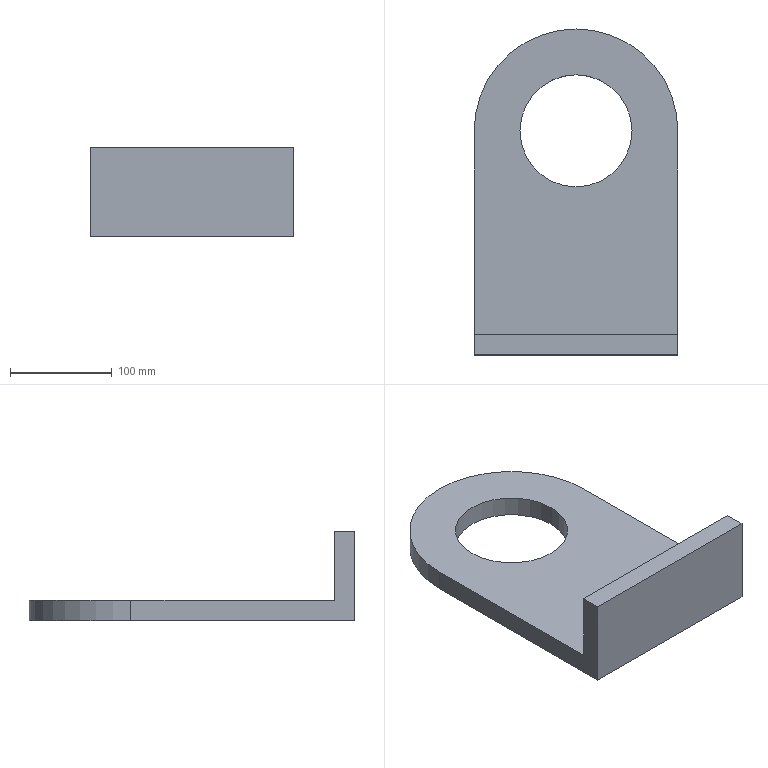Component | SolidWorks | MotorMount-1 | 1 solid | 10 faces | box 200 x 320 x 88 mm | volume 1276093 mm3 | plane 7 | cylinder 3 | commonest cylinder face diameters 110 x2 200 x1 | material 45
build123d program:
from build123d import *

# Parameters (mm, degrees)
SKETCH1_R           = 55
BOSS_EXTRUDE1_DEPTH = 20
SKETCH2_W           = 200
SKETCH2_H           = 88
BOSS_EXTRUDE2_DEPTH = 20


with BuildPart() as part:
    # Sketch1 → Boss-Extrude1 (new body)
    with BuildSketch(Plane.XY):
        with BuildLine():
            Line((-100, 0), (-100, -200))
            Line((-100, -200), (100, -200))
            Line((100, -200), (100, 0))
            ThreePointArc((100, 0), (0, 100), (-100, 0))
        make_face()
        Circle(SKETCH1_R, mode=Mode.SUBTRACT)
    extrude(amount=BOSS_EXTRUDE1_DEPTH)

    # Sketch2 → Boss-Extrude2 (add)
    with BuildSketch(Plane.XZ.offset(200)):
        with Locations((0, 44)):
            Rectangle(SKETCH2_W, SKETCH2_H)
    extrude(amount=BOSS_EXTRUDE2_DEPTH)


solid = part.part

# Placed as in the assembly
solid = solid.moved(Location((110.202, 126.699, 514.267), (0, 0, 0)))
STEP:
#1=COLOUR_RGB('',0.7922,0.8196,0.9333);
#2=FILL_AREA_STYLE_COLOUR('',#1);
#3=FILL_AREA_STYLE('',(#2));
#4=SURFACE_STYLE_FILL_AREA(#3);
#5=SURFACE_SIDE_STYLE('',(#4));
#6=SURFACE_STYLE_USAGE(.BOTH.,#5);
#7=PRESENTATION_STYLE_ASSIGNMENT((#6));
#8=CARTESIAN_POINT('',(2.173,4.988,21.034));
#9=VERTEX_POINT('',#8);
#10=CARTESIAN_POINT('',(6.504,4.988,21.034));
#11=VERTEX_POINT('',#10);
#12=CARTESIAN_POINT('',(4.339,4.988,21.034));
#13=DIRECTION('',(0.,0.,1.));
#14=DIRECTION('',(1.,0.,0.));
#15=AXIS2_PLACEMENT_3D('',#12,#13,#14);
#16=CIRCLE('',#15,2.165);
#17=EDGE_CURVE('',#9,#11,#16,.T.);
#18=ORIENTED_EDGE('',*,*,#17,.T.);
#19=CARTESIAN_POINT('',(6.504,4.988,20.247));
#20=VERTEX_POINT('',#19);
#21=CARTESIAN_POINT('',(6.504,4.988,21.034));
#22=DIRECTION('',(0.,0.,-1.));
#23=VECTOR('',#22,39.37);
#24=LINE('',#21,#23);
#25=EDGE_CURVE('',#11,#20,#24,.T.);
#26=ORIENTED_EDGE('',*,*,#25,.T.);
#27=CARTESIAN_POINT('',(2.173,4.988,20.247));
#28=VERTEX_POINT('',#27);
#29=CARTESIAN_POINT('',(4.339,4.988,20.247));
#30=DIRECTION('',(0.,0.,1.));
#31=DIRECTION('',(1.,0.,0.));
#32=AXIS2_PLACEMENT_3D('',#29,#30,#31);
#33=CIRCLE('',#32,2.165);
#34=EDGE_CURVE('',#28,#20,#33,.T.);
#35=ORIENTED_EDGE('',*,*,#34,.F.);
#36=CARTESIAN_POINT('',(2.173,4.988,21.034));
#37=DIRECTION('',(0.,0.,-1.));
#38=VECTOR('',#37,39.37);
#39=LINE('',#36,#38);
#40=EDGE_CURVE('',#9,#28,#39,.T.);
#41=ORIENTED_EDGE('',*,*,#40,.F.);
#42=EDGE_LOOP('',(#18,#26,#35,#41));
#43=FACE_OUTER_BOUND('',#42,.T.);
#44=CARTESIAN_POINT('',(4.339,4.988,21.034));
#45=DIRECTION('',(0.,0.,-1.));
#46=DIRECTION('',(-1.,0.,0.));
#47=AXIS2_PLACEMENT_3D('',#44,#45,#46);
#48=CYLINDRICAL_SURFACE('',#47,2.165);
#49=ADVANCED_FACE('',(#43),#48,.F.);
#50=CARTESIAN_POINT('',(8.276,4.988,21.034));
#51=VERTEX_POINT('',#50);
#52=CARTESIAN_POINT('',(0.4017,4.988,21.034));
#53=VERTEX_POINT('',#52);
#54=CARTESIAN_POINT('',(4.339,4.988,21.034));
#55=DIRECTION('',(0.,0.,1.));
#56=DIRECTION('',(1.,0.,0.));
#57=AXIS2_PLACEMENT_3D('',#54,#55,#56);
#58=CIRCLE('',#57,3.937);
#59=EDGE_CURVE('',#51,#53,#58,.T.);
#60=ORIENTED_EDGE('',*,*,#59,.T.);
#61=CARTESIAN_POINT('',(0.4017,-2.886,21.034));
#62=VERTEX_POINT('',#61);
#63=CARTESIAN_POINT('',(0.4017,4.988,21.034));
#64=DIRECTION('',(0.,-1.,0.));
#65=VECTOR('',#64,39.37);
#66=LINE('',#63,#65);
#67=EDGE_CURVE('',#53,#62,#66,.T.);
#68=ORIENTED_EDGE('',*,*,#67,.T.);
#69=CARTESIAN_POINT('',(8.276,-2.886,21.034));
#70=VERTEX_POINT('',#69);
#71=CARTESIAN_POINT('',(0.4017,-2.886,21.034));
#72=DIRECTION('',(1.,0.,0.));
#73=VECTOR('',#72,39.37);
#74=LINE('',#71,#73);
#75=EDGE_CURVE('',#62,#70,#74,.T.);
#76=ORIENTED_EDGE('',*,*,#75,.T.);
#77=CARTESIAN_POINT('',(8.276,-2.886,21.034));
#78=DIRECTION('',(0.,1.,0.));
#79=VECTOR('',#78,39.37);
#80=LINE('',#77,#79);
#81=EDGE_CURVE('',#70,#51,#80,.T.);
#82=ORIENTED_EDGE('',*,*,#81,.T.);
#83=EDGE_LOOP('',(#60,#68,#76,#82));
#84=FACE_OUTER_BOUND('',#83,.T.);
#85=ORIENTED_EDGE('',*,*,#17,.F.);
#86=CARTESIAN_POINT('',(4.339,4.988,21.034));
#87=DIRECTION('',(0.,0.,1.));
#88=DIRECTION('',(1.,0.,0.));
#89=AXIS2_PLACEMENT_3D('',#86,#87,#88);
#90=CIRCLE('',#89,2.165);
#91=EDGE_CURVE('',#11,#9,#90,.T.);
#92=ORIENTED_EDGE('',*,*,#91,.F.);
#93=EDGE_LOOP('',(#85,#92));
#94=FACE_BOUND('',#93,.T.);
#95=CARTESIAN_POINT('',(4.339,4.988,21.034));
#96=DIRECTION('',(0.,0.,1.));
#97=DIRECTION('',(1.,0.,0.));
#98=AXIS2_PLACEMENT_3D('',#95,#96,#97);
#99=PLANE('',#98);
#100=ADVANCED_FACE('',(#84,#94),#99,.T.);
#101=CARTESIAN_POINT('',(8.276,4.988,20.247));
#102=VERTEX_POINT('',#101);
#103=CARTESIAN_POINT('',(0.4017,4.988,20.247));
#104=VERTEX_POINT('',#103);
#105=CARTESIAN_POINT('',(4.339,4.988,20.247));
#106=DIRECTION('',(0.,0.,1.));
#107=DIRECTION('',(1.,0.,0.));
#108=AXIS2_PLACEMENT_3D('',#105,#106,#107);
#109=CIRCLE('',#108,3.937);
#110=EDGE_CURVE('',#102,#104,#109,.T.);
#111=ORIENTED_EDGE('',*,*,#110,.F.);
#112=CARTESIAN_POINT('',(8.276,-3.673,20.247));
#113=VERTEX_POINT('',#112);
#114=CARTESIAN_POINT('',(8.276,-2.886,20.247));
#115=DIRECTION('',(0.,1.,0.));
#116=VECTOR('',#115,39.37);
#117=LINE('',#114,#116);
#118=EDGE_CURVE('',#113,#102,#117,.T.);
#119=ORIENTED_EDGE('',*,*,#118,.F.);
#120=CARTESIAN_POINT('',(0.4017,-3.673,20.247));
#121=VERTEX_POINT('',#120);
#122=CARTESIAN_POINT('',(0.4017,-3.673,20.247));
#123=DIRECTION('',(1.,0.,0.));
#124=VECTOR('',#123,39.37);
#125=LINE('',#122,#124);
#126=EDGE_CURVE('',#121,#113,#125,.T.);
#127=ORIENTED_EDGE('',*,*,#126,.F.);
#128=CARTESIAN_POINT('',(0.4017,4.988,20.247));
#129=DIRECTION('',(0.,-1.,0.));
#130=VECTOR('',#129,39.37);
#131=LINE('',#128,#130);
#132=EDGE_CURVE('',#104,#121,#131,.T.);
#133=ORIENTED_EDGE('',*,*,#132,.F.);
#134=EDGE_LOOP('',(#111,#119,#127,#133));
#135=FACE_OUTER_BOUND('',#134,.T.);
#136=ORIENTED_EDGE('',*,*,#34,.T.);
#137=CARTESIAN_POINT('',(4.339,4.988,20.247));
#138=DIRECTION('',(0.,0.,1.));
#139=DIRECTION('',(1.,0.,0.));
#140=AXIS2_PLACEMENT_3D('',#137,#138,#139);
#141=CIRCLE('',#140,2.165);
#142=EDGE_CURVE('',#20,#28,#141,.T.);
#143=ORIENTED_EDGE('',*,*,#142,.T.);
#144=EDGE_LOOP('',(#136,#143));
#145=FACE_BOUND('',#144,.T.);
#146=CARTESIAN_POINT('',(4.339,4.988,20.247));
#147=DIRECTION('',(0.,0.,1.));
#148=DIRECTION('',(1.,0.,0.));
#149=AXIS2_PLACEMENT_3D('',#146,#147,#148);
#150=PLANE('',#149);
#151=ADVANCED_FACE('',(#135,#145),#150,.F.);
#152=ORIENTED_EDGE('',*,*,#110,.T.);
#153=CARTESIAN_POINT('',(0.4017,4.988,21.034));
#154=DIRECTION('',(0.,0.,-1.));
#155=VECTOR('',#154,39.37);
#156=LINE('',#153,#155);
#157=EDGE_CURVE('',#53,#104,#156,.T.);
#158=ORIENTED_EDGE('',*,*,#157,.F.);
#159=ORIENTED_EDGE('',*,*,#59,.F.);
#160=CARTESIAN_POINT('',(8.276,4.988,21.034));
#161=DIRECTION('',(0.,0.,-1.));
#162=VECTOR('',#161,39.37);
#163=LINE('',#160,#162);
#164=EDGE_CURVE('',#51,#102,#163,.T.);
#165=ORIENTED_EDGE('',*,*,#164,.T.);
#166=EDGE_LOOP('',(#152,#158,#159,#165));
#167=FACE_OUTER_BOUND('',#166,.T.);
#168=CARTESIAN_POINT('',(4.339,4.988,21.034));
#169=DIRECTION('',(0.,0.,-1.));
#170=DIRECTION('',(-1.,0.,0.));
#171=AXIS2_PLACEMENT_3D('',#168,#169,#170);
#172=CYLINDRICAL_SURFACE('',#171,3.937);
#173=ADVANCED_FACE('',(#167),#172,.T.);
#174=ORIENTED_EDGE('',*,*,#132,.T.);
#175=CARTESIAN_POINT('',(0.4017,-3.673,23.711));
#176=VERTEX_POINT('',#175);
#177=CARTESIAN_POINT('',(0.4017,-3.673,20.247));
#178=DIRECTION('',(0.,0.,-1.));
#179=VECTOR('',#178,39.37);
#180=LINE('',#177,#179);
#181=EDGE_CURVE('',#176,#121,#180,.T.);
#182=ORIENTED_EDGE('',*,*,#181,.F.);
#183=CARTESIAN_POINT('',(0.4017,-2.886,23.711));
#184=VERTEX_POINT('',#183);
#185=CARTESIAN_POINT('',(0.4017,-3.673,23.711));
#186=DIRECTION('',(0.,1.,0.));
#187=VECTOR('',#186,39.37);
#188=LINE('',#185,#187);
#189=EDGE_CURVE('',#176,#184,#188,.T.);
#190=ORIENTED_EDGE('',*,*,#189,.T.);
#191=CARTESIAN_POINT('',(0.4017,-2.886,20.247));
#192=DIRECTION('',(0.,0.,-1.));
#193=VECTOR('',#192,39.37);
#194=LINE('',#191,#193);
#195=EDGE_CURVE('',#184,#62,#194,.T.);
#196=ORIENTED_EDGE('',*,*,#195,.T.);
#197=ORIENTED_EDGE('',*,*,#67,.F.);
#198=ORIENTED_EDGE('',*,*,#157,.T.);
#199=EDGE_LOOP('',(#174,#182,#190,#196,#197,#198));
#200=FACE_OUTER_BOUND('',#199,.T.);
#201=CARTESIAN_POINT('',(0.4017,4.988,21.034));
#202=DIRECTION('',(1.,0.,0.));
#203=DIRECTION('',(-0.,1.,0.));
#204=AXIS2_PLACEMENT_3D('',#201,#202,#203);
#205=PLANE('',#204);
#206=ADVANCED_FACE('',(#200),#205,.F.);
#207=ORIENTED_EDGE('',*,*,#118,.T.);
#208=ORIENTED_EDGE('',*,*,#164,.F.);
#209=ORIENTED_EDGE('',*,*,#81,.F.);
#210=CARTESIAN_POINT('',(8.276,-2.886,23.711));
#211=VERTEX_POINT('',#210);
#212=CARTESIAN_POINT('',(8.276,-2.886,20.247));
#213=DIRECTION('',(0.,0.,1.));
#214=VECTOR('',#213,39.37);
#215=LINE('',#212,#214);
#216=EDGE_CURVE('',#70,#211,#215,.T.);
#217=ORIENTED_EDGE('',*,*,#216,.T.);
#218=CARTESIAN_POINT('',(8.276,-3.673,23.711));
#219=VERTEX_POINT('',#218);
#220=CARTESIAN_POINT('',(8.276,-3.673,23.711));
#221=DIRECTION('',(0.,1.,0.));
#222=VECTOR('',#221,39.37);
#223=LINE('',#220,#222);
#224=EDGE_CURVE('',#219,#211,#223,.T.);
#225=ORIENTED_EDGE('',*,*,#224,.F.);
#226=CARTESIAN_POINT('',(8.276,-3.673,20.247));
#227=DIRECTION('',(0.,0.,1.));
#228=VECTOR('',#227,39.37);
#229=LINE('',#226,#228);
#230=EDGE_CURVE('',#113,#219,#229,.T.);
#231=ORIENTED_EDGE('',*,*,#230,.F.);
#232=EDGE_LOOP('',(#207,#208,#209,#217,#225,#231));
#233=FACE_OUTER_BOUND('',#232,.T.);
#234=CARTESIAN_POINT('',(8.276,-2.886,21.034));
#235=DIRECTION('',(-1.,0.,0.));
#236=DIRECTION('',(-0.,-1.,0.));
#237=AXIS2_PLACEMENT_3D('',#234,#235,#236);
#238=PLANE('',#237);
#239=ADVANCED_FACE('',(#233),#238,.F.);
#240=ORIENTED_EDGE('',*,*,#25,.F.);
#241=ORIENTED_EDGE('',*,*,#91,.T.);
#242=ORIENTED_EDGE('',*,*,#40,.T.);
#243=ORIENTED_EDGE('',*,*,#142,.F.);
#244=EDGE_LOOP('',(#240,#241,#242,#243));
#245=FACE_OUTER_BOUND('',#244,.T.);
#246=CARTESIAN_POINT('',(4.339,4.988,21.034));
#247=DIRECTION('',(0.,0.,-1.));
#248=DIRECTION('',(-1.,0.,0.));
#249=AXIS2_PLACEMENT_3D('',#246,#247,#248);
#250=CYLINDRICAL_SURFACE('',#249,2.165);
#251=ADVANCED_FACE('',(#245),#250,.F.);
#252=ORIENTED_EDGE('',*,*,#75,.F.);
#253=ORIENTED_EDGE('',*,*,#195,.F.);
#254=CARTESIAN_POINT('',(0.4017,-2.886,23.711));
#255=DIRECTION('',(-1.,0.,0.));
#256=VECTOR('',#255,39.37);
#257=LINE('',#254,#256);
#258=EDGE_CURVE('',#211,#184,#257,.T.);
#259=ORIENTED_EDGE('',*,*,#258,.F.);
#260=ORIENTED_EDGE('',*,*,#216,.F.);
#261=EDGE_LOOP('',(#252,#253,#259,#260));
#262=FACE_OUTER_BOUND('',#261,.T.);
#263=CARTESIAN_POINT('',(4.339,-2.886,20.247));
#264=DIRECTION('',(0.,1.,0.));
#265=DIRECTION('',(0.,0.,1.));
#266=AXIS2_PLACEMENT_3D('',#263,#264,#265);
#267=PLANE('',#266);
#268=ADVANCED_FACE('',(#262),#267,.T.);
#269=ORIENTED_EDGE('',*,*,#258,.T.);
#270=ORIENTED_EDGE('',*,*,#189,.F.);
#271=CARTESIAN_POINT('',(0.4017,-3.673,23.711));
#272=DIRECTION('',(-1.,0.,0.));
#273=VECTOR('',#272,39.37);
#274=LINE('',#271,#273);
#275=EDGE_CURVE('',#219,#176,#274,.T.);
#276=ORIENTED_EDGE('',*,*,#275,.F.);
#277=ORIENTED_EDGE('',*,*,#224,.T.);
#278=EDGE_LOOP('',(#269,#270,#276,#277));
#279=FACE_OUTER_BOUND('',#278,.T.);
#280=CARTESIAN_POINT('',(0.4017,-3.673,23.711));
#281=DIRECTION('',(0.,0.,-1.));
#282=DIRECTION('',(-1.,0.,0.));
#283=AXIS2_PLACEMENT_3D('',#280,#281,#282);
#284=PLANE('',#283);
#285=ADVANCED_FACE('',(#279),#284,.F.);
#286=ORIENTED_EDGE('',*,*,#181,.T.);
#287=ORIENTED_EDGE('',*,*,#126,.T.);
#288=ORIENTED_EDGE('',*,*,#230,.T.);
#289=ORIENTED_EDGE('',*,*,#275,.T.);
#290=EDGE_LOOP('',(#286,#287,#288,#289));
#291=FACE_OUTER_BOUND('',#290,.T.);
#292=CARTESIAN_POINT('',(4.339,-3.673,20.247));
#293=DIRECTION('',(0.,1.,0.));
#294=DIRECTION('',(0.,0.,1.));
#295=AXIS2_PLACEMENT_3D('',#292,#293,#294);
#296=PLANE('',#295);
#297=ADVANCED_FACE('',(#291),#296,.F.);
#298=CLOSED_SHELL('',(#49,#100,#151,#173,#206,#239,#251,#268,#285,#297));
#299=MANIFOLD_SOLID_BREP('',#298);
#300=STYLED_ITEM('',(#7),#299);
#301=(LENGTH_UNIT()NAMED_UNIT(*)SI_UNIT($,.METRE.));
#302=LENGTH_MEASURE_WITH_UNIT(LENGTH_MEASURE(0.0254),#301);
#303=DIMENSIONAL_EXPONENTS(1.,0.,0.,0.,0.,0.,0.);
#304=(CONVERSION_BASED_UNIT('',#302)LENGTH_UNIT()NAMED_UNIT(#303));
#305=UNCERTAINTY_MEASURE_WITH_UNIT(LENGTH_MEASURE(0.00001),#304,'','');
#306=(NAMED_UNIT(*)PLANE_ANGLE_UNIT()SI_UNIT($,.RADIAN.));
#307=(NAMED_UNIT(*)SI_UNIT($,.STERADIAN.)SOLID_ANGLE_UNIT());
#308=(GEOMETRIC_REPRESENTATION_CONTEXT(3)GLOBAL_UNCERTAINTY_ASSIGNED_CONTEXT((#305))GLOBAL_UNIT_ASSIGNED_CONTEXT((#304,#306,#307))REPRESENTATION_CONTEXT('',''));
#309=MECHANICAL_DESIGN_GEOMETRIC_PRESENTATION_REPRESENTATION('',(#300),#308);
#310=PRESENTATION_LAYER_ASSIGNMENT('','',(#300));
#311=CARTESIAN_POINT('',(0.,0.,0.));
#312=DIRECTION('',(0.,0.,1.));
#313=DIRECTION('',(1.,0.,0.));
#314=AXIS2_PLACEMENT_3D('',#311,#312,#313);
#315=(LENGTH_UNIT()NAMED_UNIT(*)SI_UNIT($,.METRE.));
#316=LENGTH_MEASURE_WITH_UNIT(LENGTH_MEASURE(0.0254),#315);
#317=DIMENSIONAL_EXPONENTS(1.,0.,0.,0.,0.,0.,0.);
#318=(CONVERSION_BASED_UNIT('',#316)LENGTH_UNIT()NAMED_UNIT(#317));
#319=UNCERTAINTY_MEASURE_WITH_UNIT(LENGTH_MEASURE(0.00001),#318,'','');
#320=(NAMED_UNIT(*)PLANE_ANGLE_UNIT()SI_UNIT($,.RADIAN.));
#321=(NAMED_UNIT(*)SI_UNIT($,.STERADIAN.)SOLID_ANGLE_UNIT());
#322=(GEOMETRIC_REPRESENTATION_CONTEXT(3)GLOBAL_UNCERTAINTY_ASSIGNED_CONTEXT((#319))GLOBAL_UNIT_ASSIGNED_CONTEXT((#318,#320,#321))REPRESENTATION_CONTEXT('',''));
#323=ADVANCED_BREP_SHAPE_REPRESENTATION('',(#299,#314),#322);